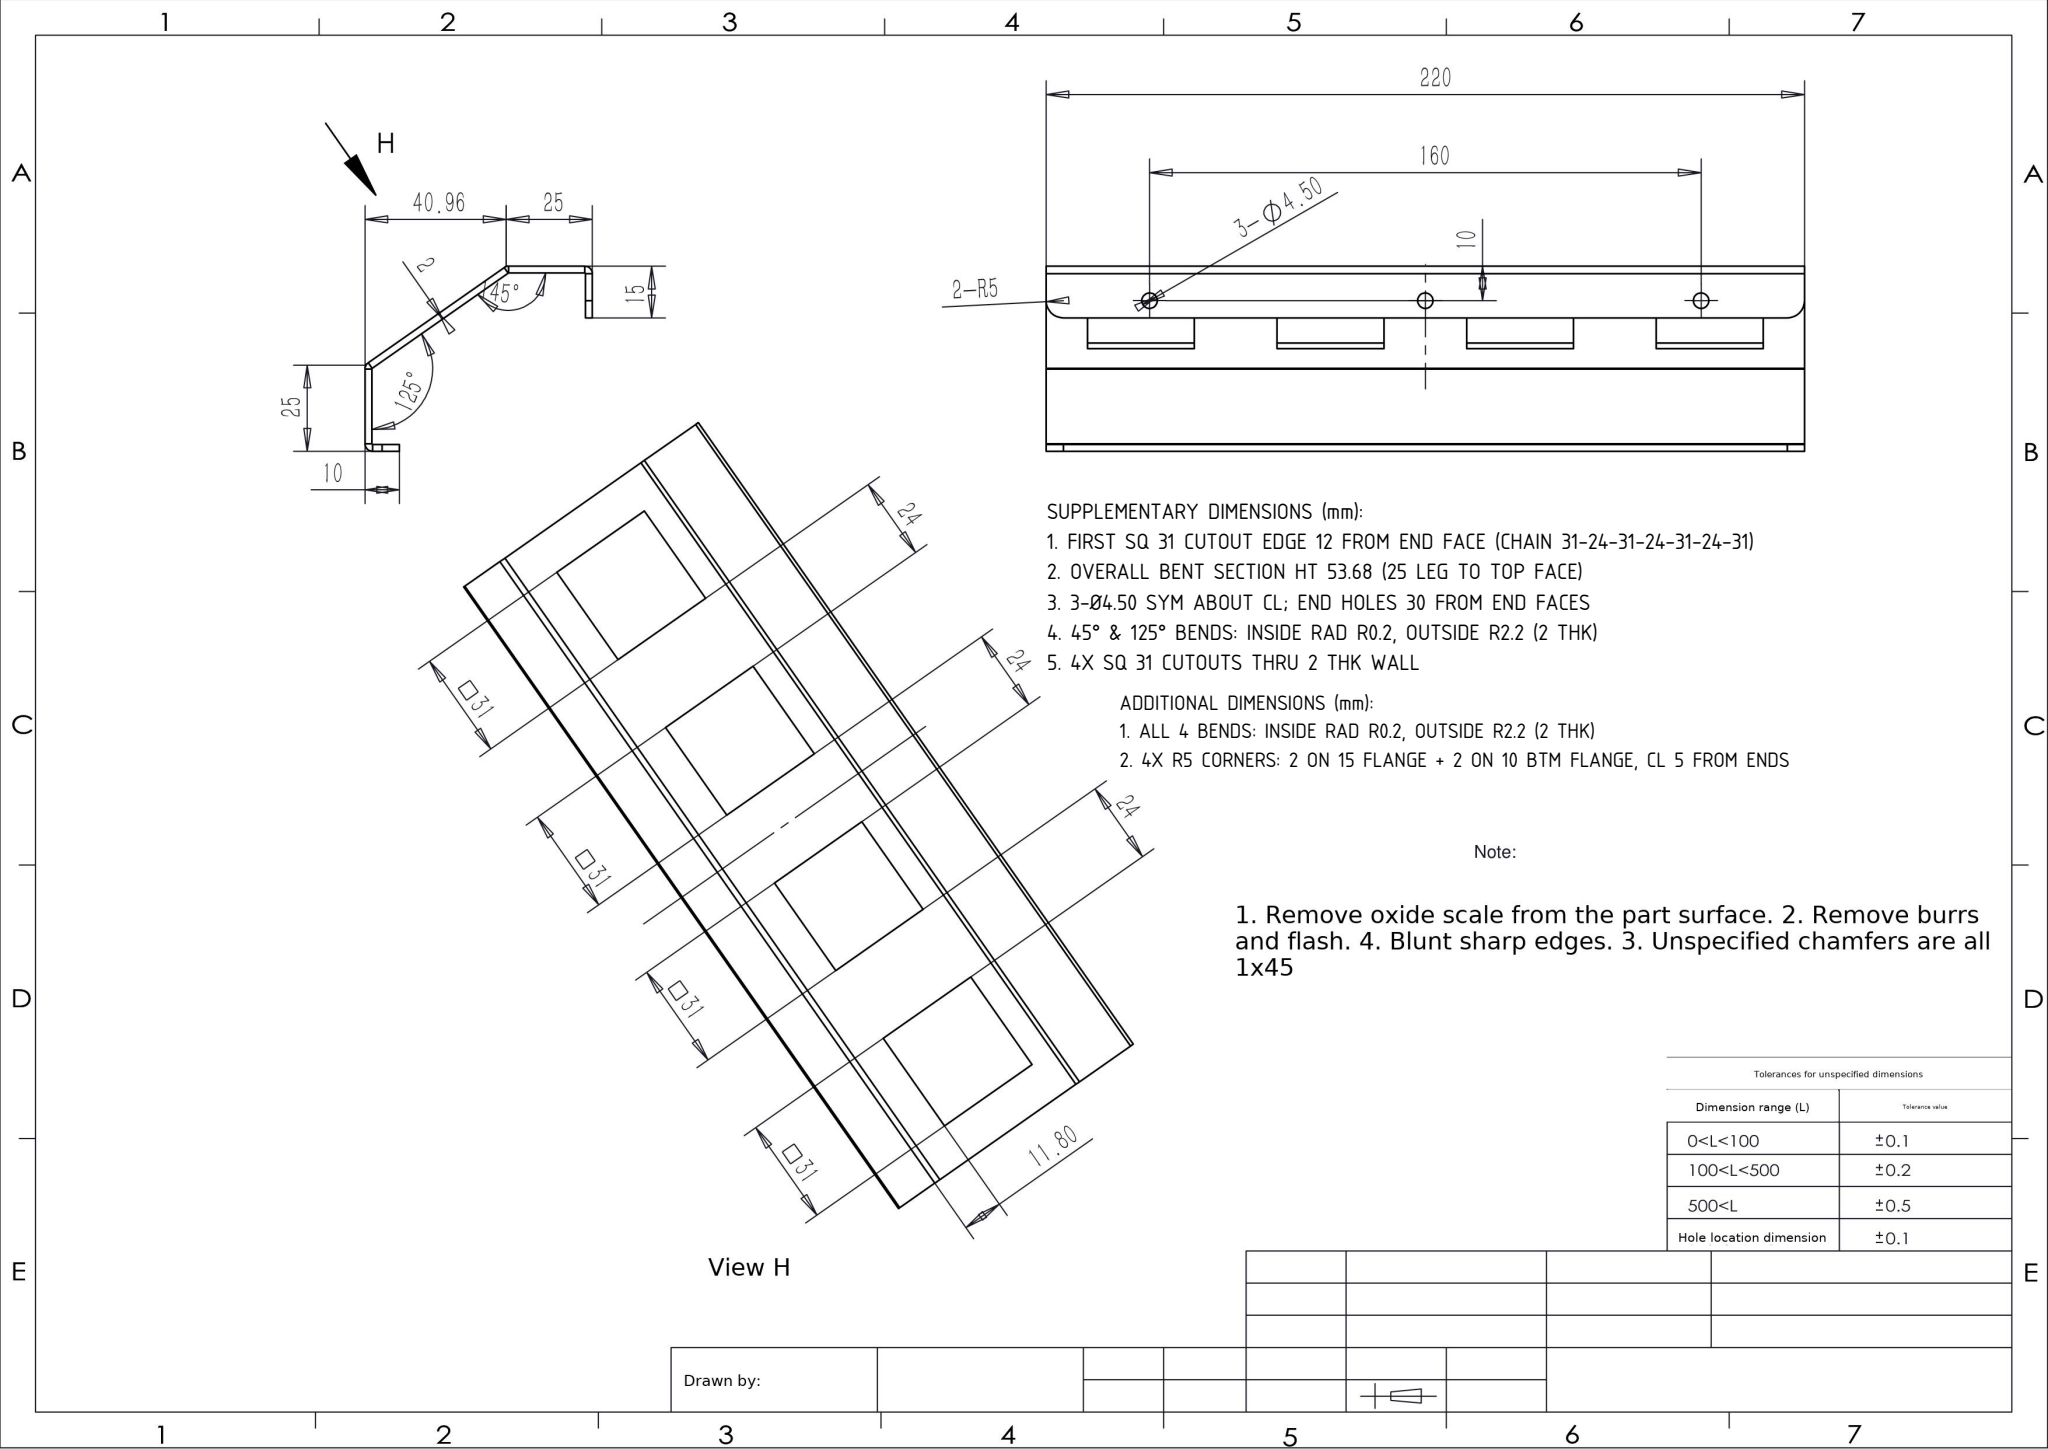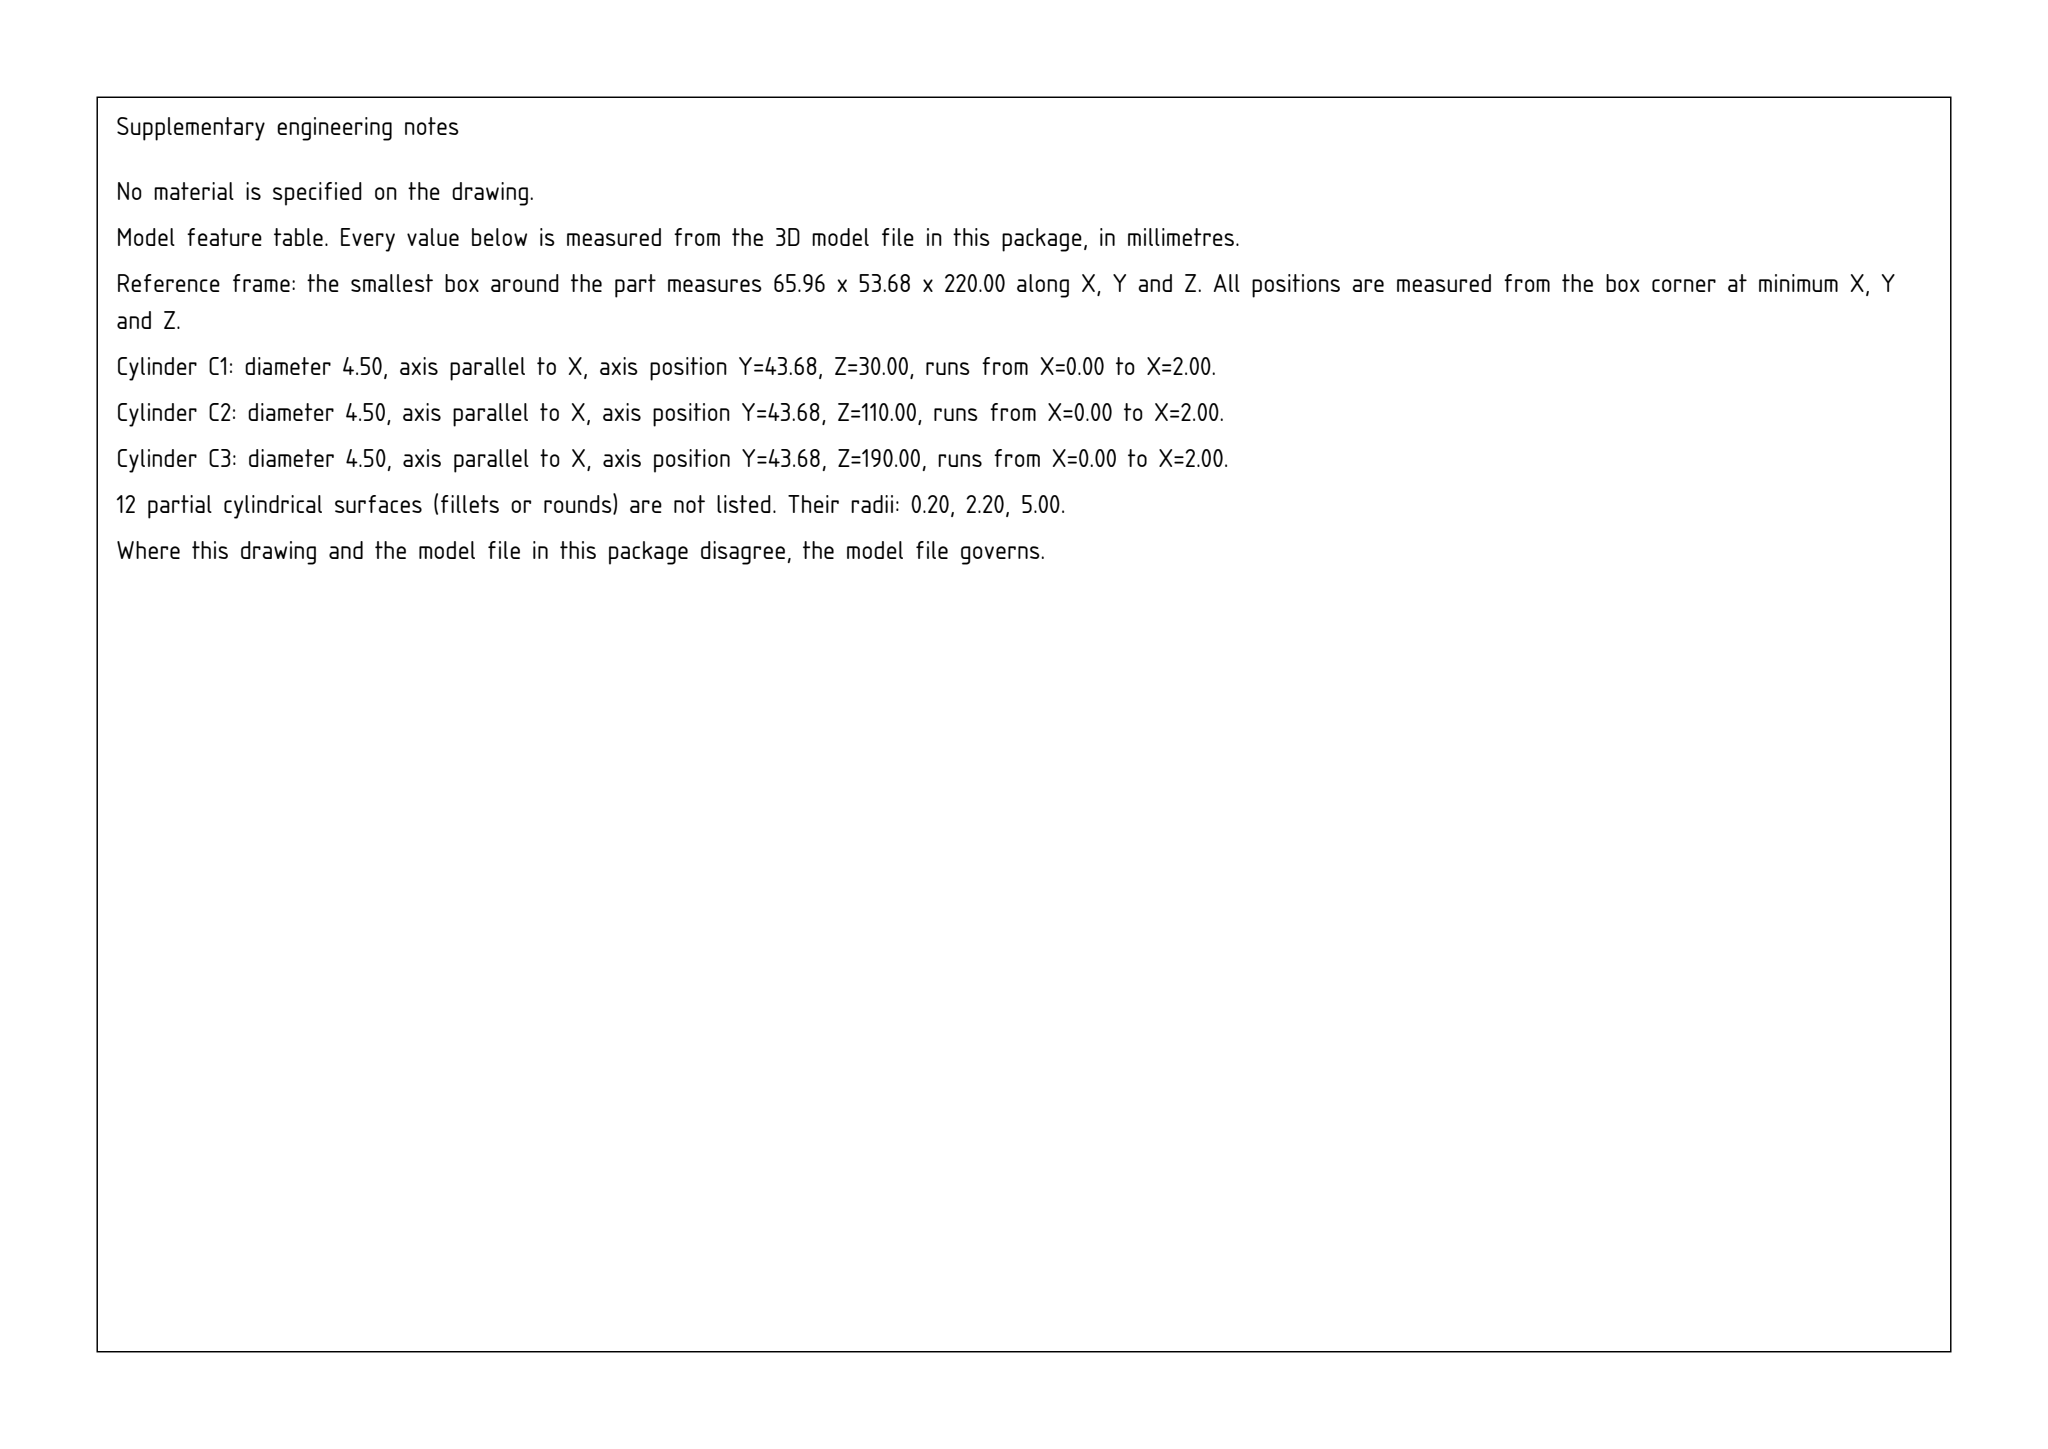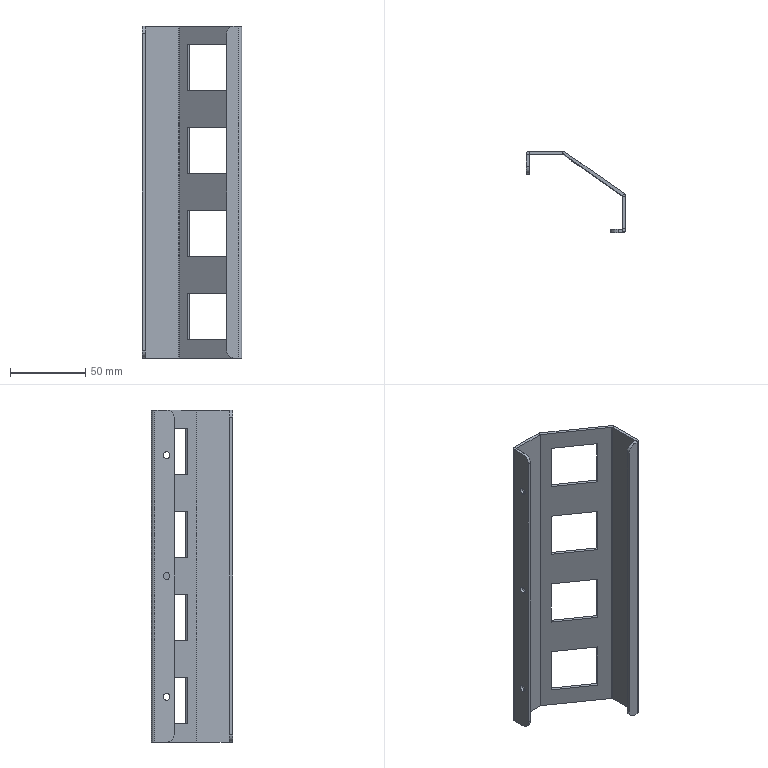Part | SolidWorks | mm | 1 solid | 64 faces | box 65.96 x 53.68 x 220 mm | volume 44172 mm3 | plane 46 | cylinder 18 | commonest cylinder face diameters 4.5 x6 4.4 x4 0.4 x4 10 x4